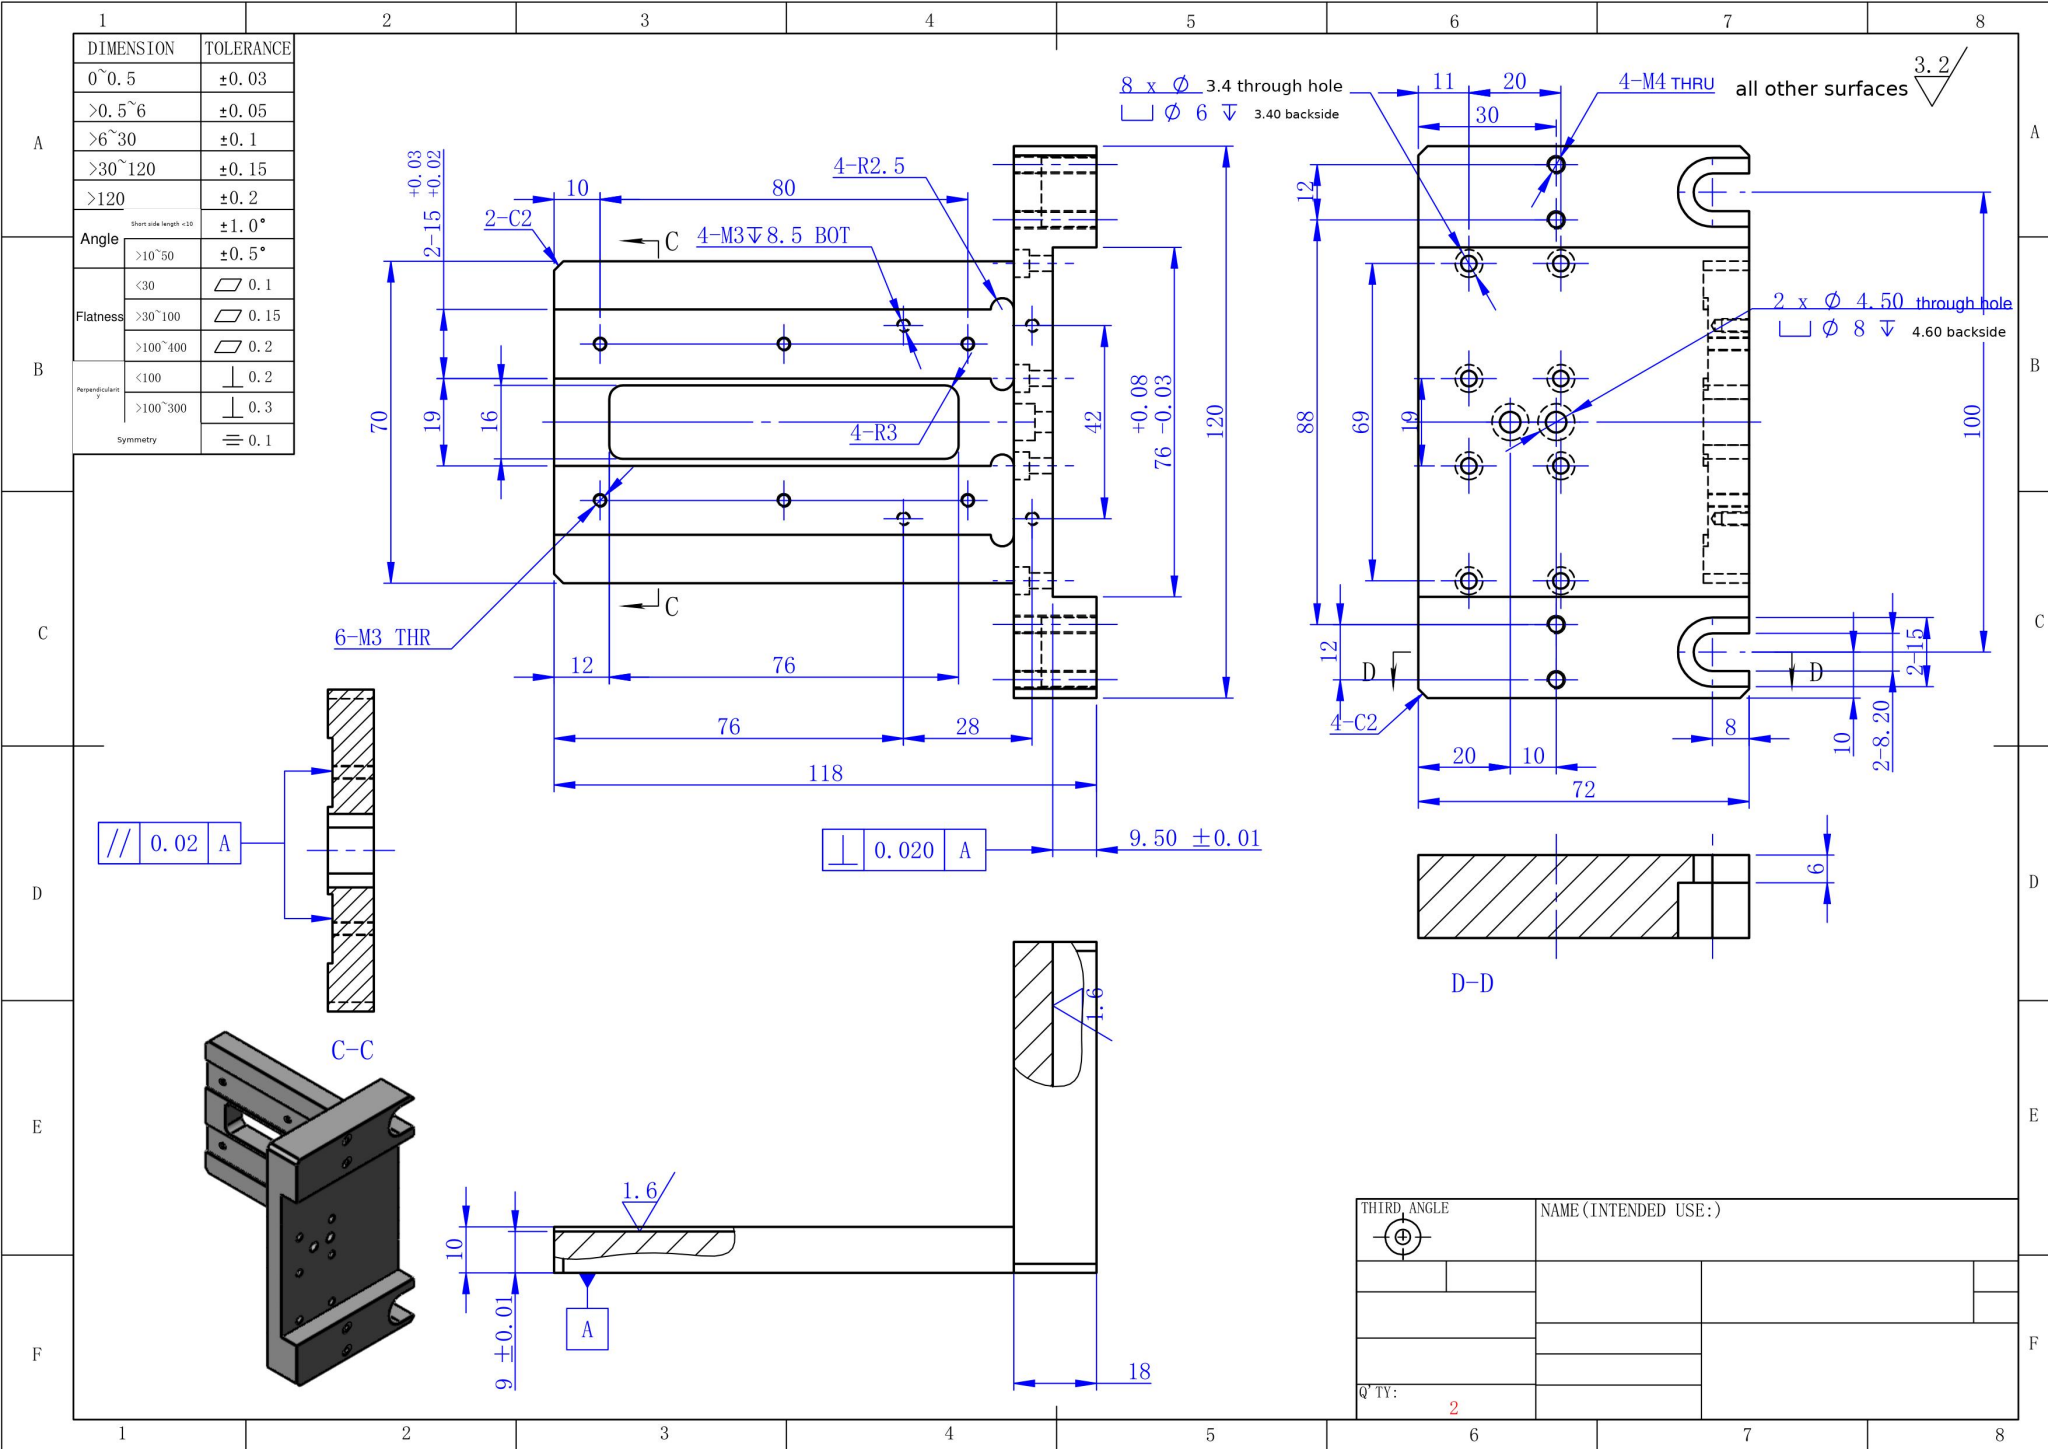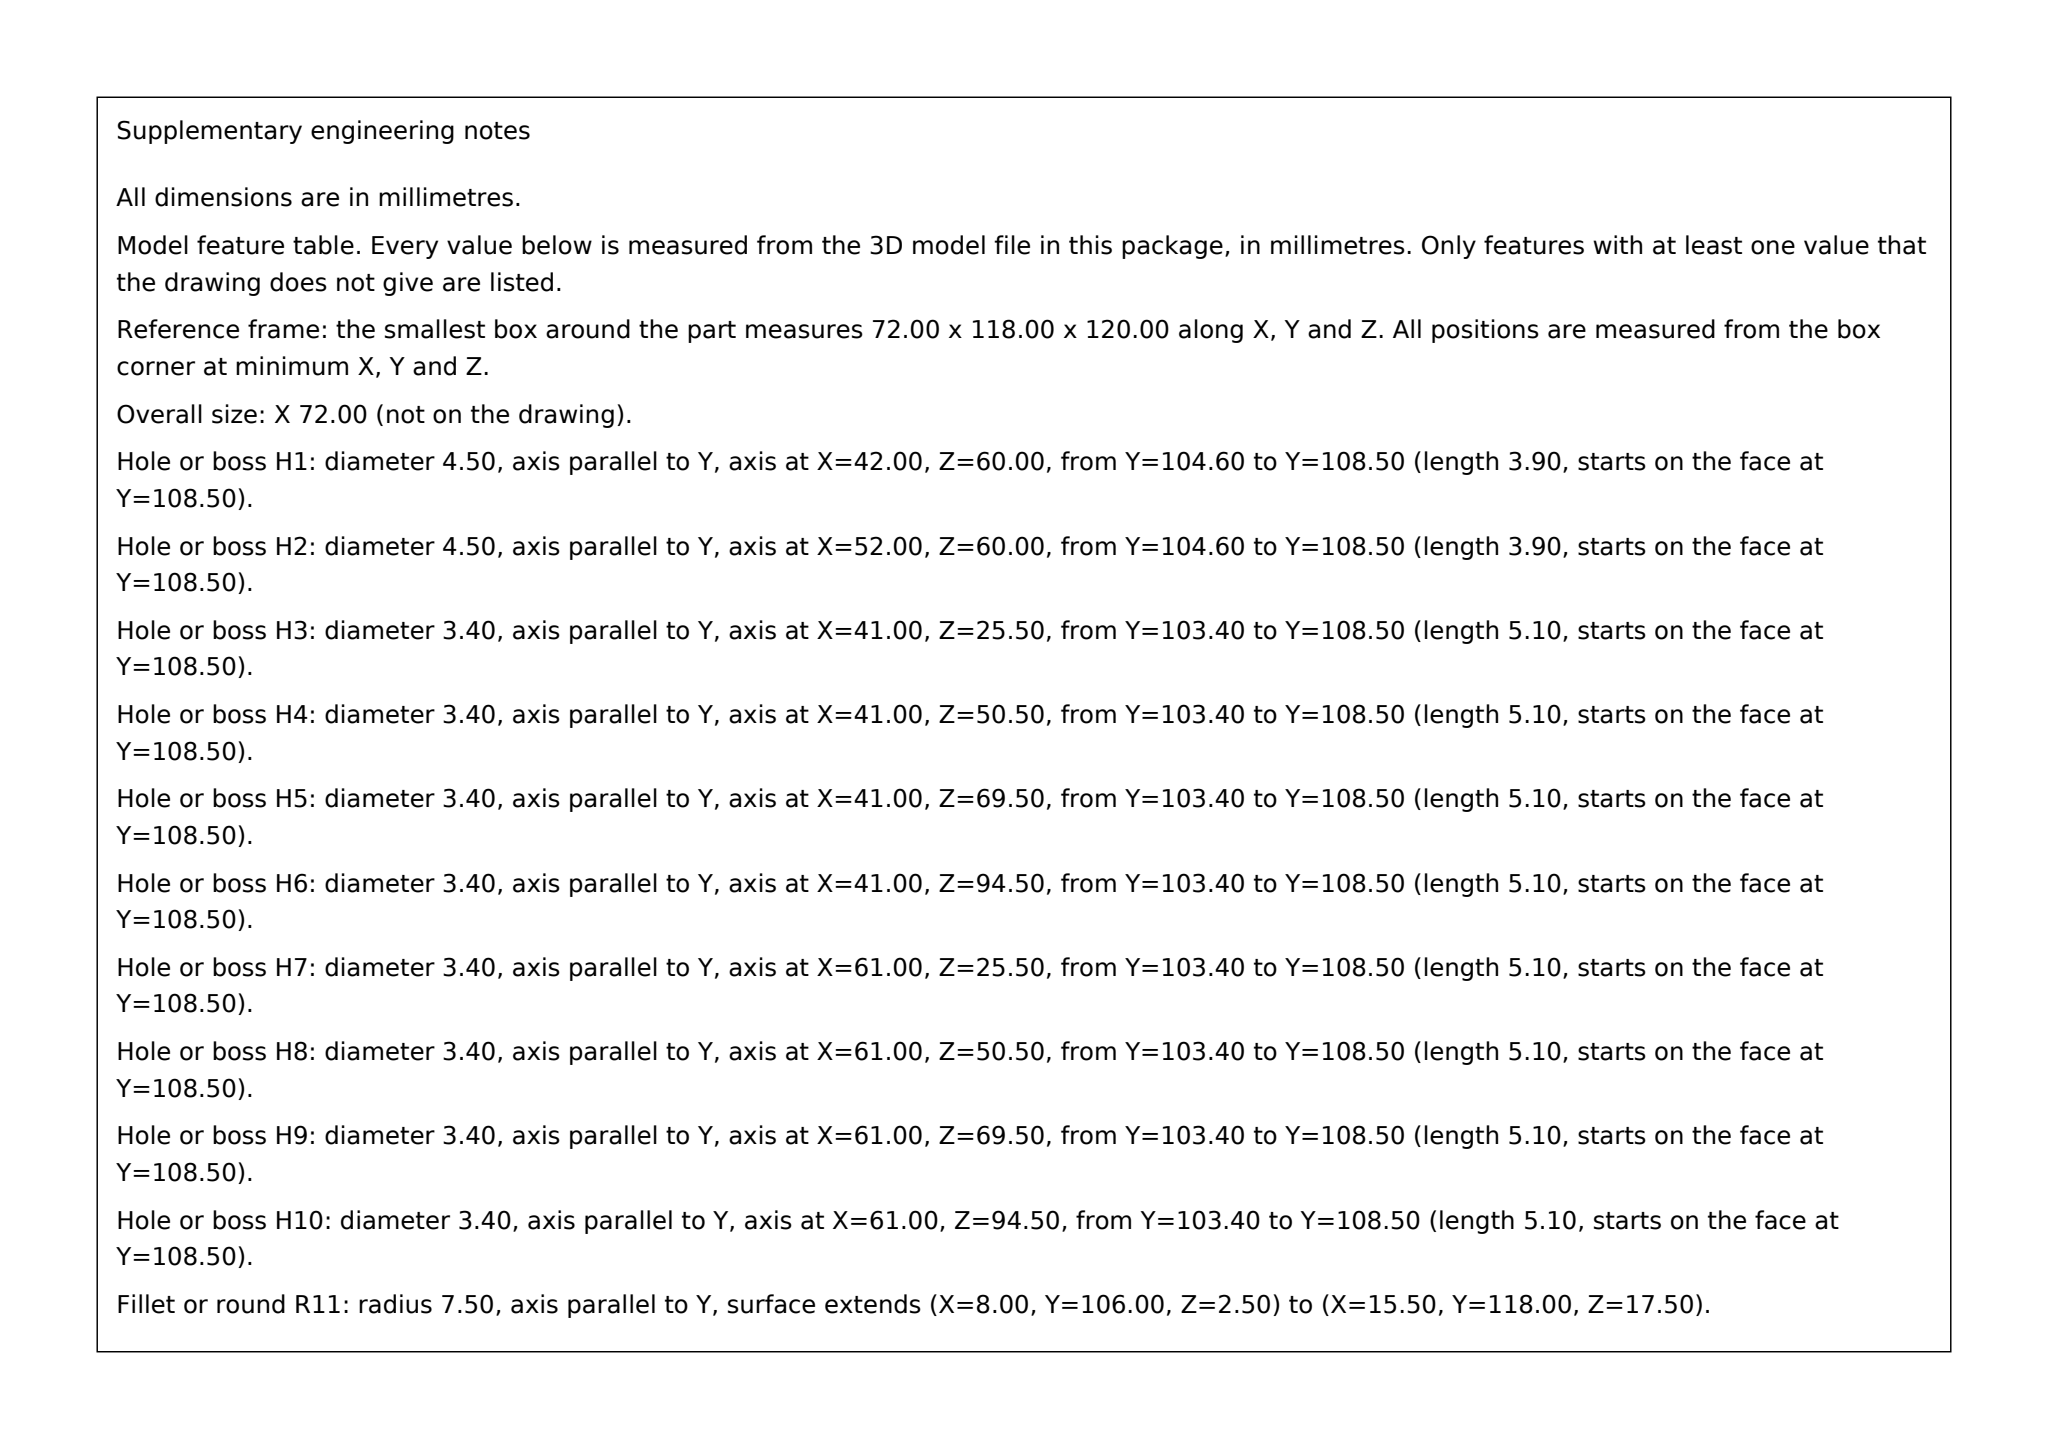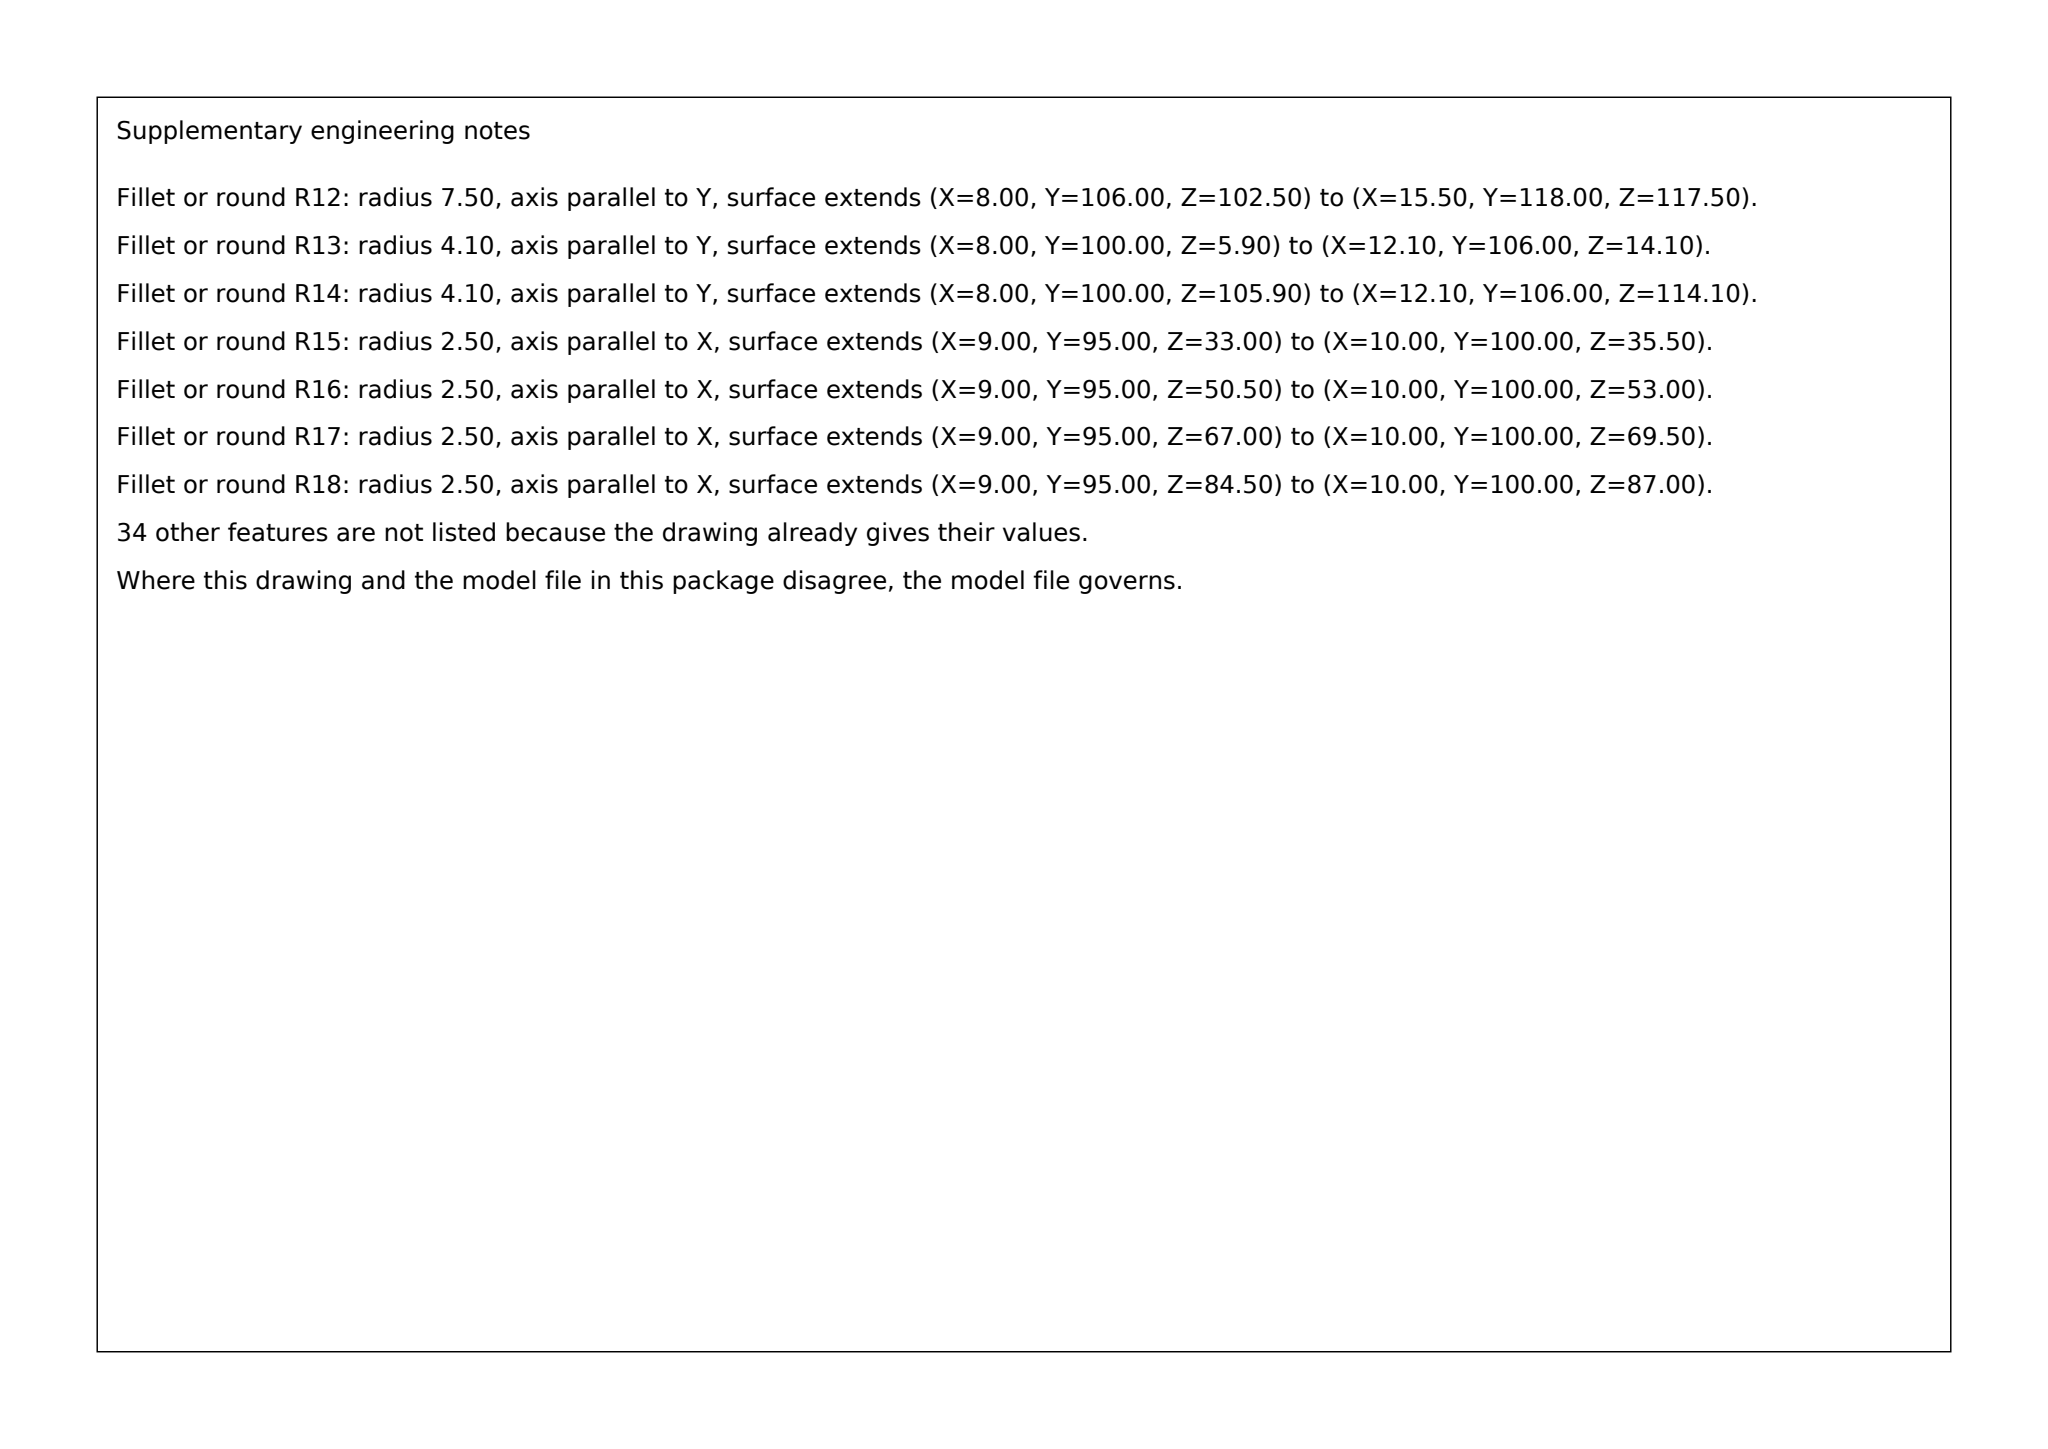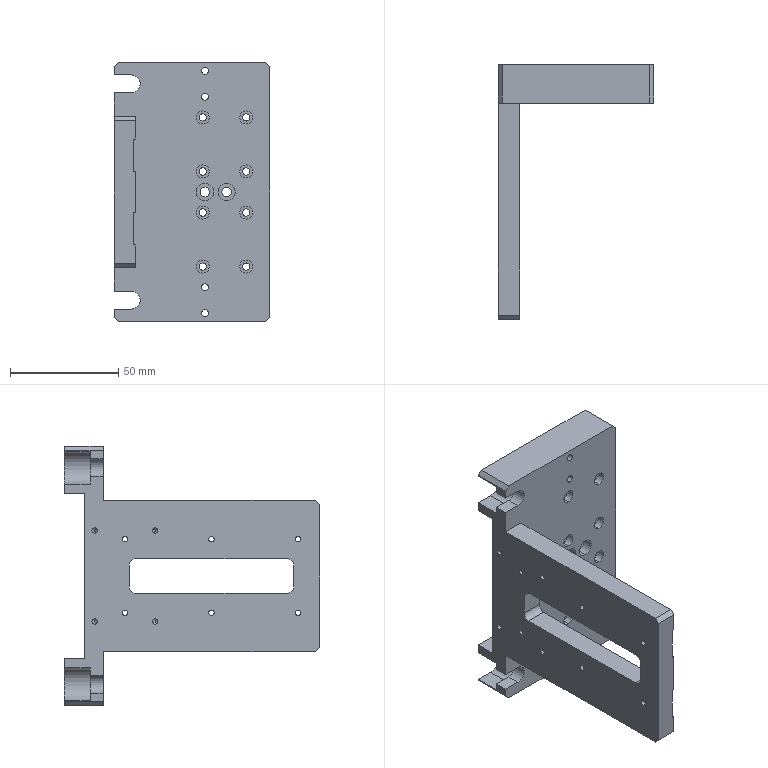Part | SolidWorks | mm | 1 solid | 142 faces | box 72 x 118 x 120 mm | volume 149366 mm3 | cylinder 80 | plane 54 | cone 8 | commonest cylinder face diameters 6 x20 2.5 x20 3.4 x16 3.3 x8 8 x4 4.5 x4 5 x4 8.2 x2
build123d program:
from build123d import *

# Parameters (mm, degrees)
BOSS_EXTRUDE1_DEPTH                                  = 35
SKETCH2_W                                            = 72
SKETCH2_H                                            = 18
BOSS_EXTRUDE2_DEPTH                                  = 25
SKETCH3_W                                            = 16
SKETCH3_H                                            = 76
CUT_EXTRUDE1_DEPTH                                   = 56
FILLET1_R                                            = 3
SKETCH9_W                                            = 21.47
SKETCH9_H                                            = 15
SKETCH9_W_2                                          = 23.046
CUT_EXTRUDE3_DEPTH                                   = 100
SKETCH10_R                                           = 2.5
CUT_EXTRUDE4_DEPTH                                   = 1
M3_TAPPED_HOLE1_D                                    = 2.5
M3_TAPPED_HOLE2_D                                    = 2.5
M3_TAPPED_HOLE2_DEPTH                                = 7.5
M3_TAPPED_HOLE2_TIP                                  = 0.7511
M4_TAPPED_HOLE2_D                                    = 3.3
HOLE_SIZE_ACCORDING_TO_THE_TYPE_OF_HEXAG_D           = 3.4
HOLE_SIZE_ACCORDING_TO_THE_TYPE_OF_HEXAG_CBORE_D     = 6
HOLE_SIZE_ACCORDING_TO_THE_TYPE_OF_HEXAG_CBORE_DEPTH = 3.4
CUT_EXTRUDE6_REACH                                   = 152.692
CUT_EXTRUDE7_DEPTH                                   = 12
CHAMFER1_SIZE                                        = 2
SKETCH23_W                                           = 76
SKETCH23_H                                           = 13.599
CUT_EXTRUDE9_DEPTH                                   = 151.692
HOLE_SIZE_ACCORDING_TO_THE_TYPE_OF_H_2_D             = 4.5
HOLE_SIZE_ACCORDING_TO_THE_TYPE_OF_H_2_CBORE_D       = 8
HOLE_SIZE_ACCORDING_TO_THE_TYPE_OF_H_2_CBORE_DEPTH   = 4.6


with BuildPart() as part:
    # Sketch1 → Boss-Extrude1 (new, symmetric)
    with BuildSketch(Plane.XY):
        Polygon((0, 0), (0, 110), (72, 110), (72, 100), (10, 100), (10, 0), align=None)
    extrude(amount=BOSS_EXTRUDE1_DEPTH, both=True)

    # Sketch2 → Boss-Extrude2 (add)
    with BuildSketch(Plane(origin=(0, 0, -35), x_dir=(-1, 0, 0), z_dir=(0, 0, -1))):
        with Locations((-36, 109)):
            Rectangle(SKETCH2_W, SKETCH2_H)
    boss_extrude2 = extrude(amount=BOSS_EXTRUDE2_DEPTH)

    # Sketch3 → Cut-Extrude1 (cut)
    with BuildSketch(Plane.ZY):
        with Locations((0, 50)):
            Rectangle(SKETCH3_W, SKETCH3_H)
    extrude(amount=-CUT_EXTRUDE1_DEPTH, mode=Mode.SUBTRACT)

    # Fillet1
    fillet1_edges = [part.edges().sort_by_distance(p)[0] for p in [
        (5, 88, 8),
        (5, 12, 8),
        (5, 12, -8),
        (5, 88, -8),
    ]]
    fillet(fillet1_edges, radius=FILLET1_R)

    # Sketch9 → Cut-Extrude3 (cut)
    with BuildSketch(Plane.XZ):
        with Locations((19.735, 17)):
            Rectangle(SKETCH9_W, SKETCH9_H)
        with Locations((20.523, -17)):
            Rectangle(SKETCH9_W_2, SKETCH9_H)
    extrude(amount=-CUT_EXTRUDE3_DEPTH, mode=Mode.SUBTRACT)

    # Sketch10 → Cut-Extrude4 (cut)
    with BuildSketch(Plane(origin=(10, 0, 0), x_dir=(0, 0, -1), z_dir=(1, 0, 0))):
        with Locations((-24.5, 97.5)):
            Circle(SKETCH10_R)
        with Locations((-9.5, 97.5)):
            Circle(SKETCH10_R)
        with Locations((9.5, 97.5)):
            Circle(SKETCH10_R)
        with Locations((24.5, 97.5)):
            Circle(SKETCH10_R)
    extrude(amount=-CUT_EXTRUDE4_DEPTH, mode=Mode.SUBTRACT)

    # M3 Tapped Hole1 (through all)
    with Locations(Plane(origin=(9, 0, 0), x_dir=(0, 0, -1), z_dir=(1, 0, 0))):
        with Locations((-17, 90), (17, 90), (17, 50), (-17, 50), (-17, 10), (17, 10)):
            Hole(M3_TAPPED_HOLE1_D / 2)

    # M3 Tapped Hole2
    with Locations(Plane.ZY):
        with Locations((21, 104), (21, 76), (-21, 104), (-21, 76)):
            Hole(M3_TAPPED_HOLE2_D / 2, depth=M3_TAPPED_HOLE2_DEPTH)
            with Locations((0, 0, -(M3_TAPPED_HOLE2_DEPTH + M3_TAPPED_HOLE2_TIP / 2))):  # 118° drill point
                Cone(0, M3_TAPPED_HOLE2_D / 2, M3_TAPPED_HOLE2_TIP, mode=Mode.SUBTRACT)

    # M4 Tapped Hole2 (through all)
    with Locations(Plane(origin=(6.733, 118, -4.955), x_dir=(1, 0, 0), z_dir=(0, 1, 0))):
        with Locations((35.267, 51.045), (35.267, 39.045)):
            m4_tapped_hole2 = Hole(M4_TAPPED_HOLE2_D / 2)

    # Mirror1: Boss-Extrude2, M4 Tapped Hole2 across plane
    add(boss_extrude2.mirror(Plane.XY))
    add(m4_tapped_hole2.mirror(Plane.XY), mode=Mode.SUBTRACT)

    # Hole Size according to the type of hexag (through all)
    with Locations(Plane(origin=(0, 100, 0), x_dir=(-1, 0, 0), z_dir=(0, -1, 0))):
        with Locations((-41, 34.5), (-61, 34.5), (-41, 9.5), (-61, 9.5), (-41, -9.5), (-41, -34.5), (-61, -34.5), (-61, -9.5)):
            CounterBoreHole(HOLE_SIZE_ACCORDING_TO_THE_TYPE_OF_HEXAG_D / 2, HOLE_SIZE_ACCORDING_TO_THE_TYPE_OF_HEXAG_CBORE_D / 2, HOLE_SIZE_ACCORDING_TO_THE_TYPE_OF_HEXAG_CBORE_DEPTH)

    # Sketch20 → Cut-Extrude6 (cut, up to next)
    with BuildSketch(Plane(origin=(0, 118, 0), x_dir=(1, 0, 0), z_dir=(0, 1, 0)), mode=Mode.PRIVATE) as cut_extrude6_sk1:
        with BuildLine():
            Line((8, 45.9), (0, 45.9))
            ThreePointArc((0, 45.9), (-4.1, 50), (0, 54.1))
            Line((0, 54.1), (8, 54.1))
            ThreePointArc((8, 54.1), (12.1, 50), (8, 45.9))
        make_face()
    cut_extrude6_tool1 = extrude(cut_extrude6_sk1.sketch, amount=-CUT_EXTRUDE6_REACH, mode=Mode.PRIVATE) & part.part
    cut_extrude6 = cut_extrude6_tool1.solids().sort_by_distance((4, 118, -50))[0]
    add(cut_extrude6, mode=Mode.SUBTRACT)

    # Sketch21 → Cut-Extrude7 (cut)
    with BuildSketch(Plane(origin=(0, 118, 0), x_dir=(1, 0, 0), z_dir=(0, 1, 0))):
        with BuildLine():
            Line((8, 42.5), (0, 42.5))
            ThreePointArc((0, 42.5), (-7.5, 50), (0, 57.5))
            Line((0, 57.5), (8, 57.5))
            ThreePointArc((8, 57.5), (15.5, 50), (8, 42.5))
        make_face()
    cut_extrude7 = extrude(amount=-CUT_EXTRUDE7_DEPTH, mode=Mode.SUBTRACT)

    # Chamfer1
    chamfer1_edges = [part.edges().sort_by_distance(p)[0] for p in [
        (72, 109, -60),
        (72, 109, 60),
        (0, 109, 60),
        (0, 109, -60),
        (5, 0, 35),
        (5, 0, -35),
    ]]
    chamfer(chamfer1_edges, length=CHAMFER1_SIZE)

    # Sketch23 → Cut-Extrude9 (cut, through all)
    with BuildSketch(Plane.ZY):
        with Locations((0, 115.299)):
            Rectangle(SKETCH23_W, SKETCH23_H)
    extrude(amount=-CUT_EXTRUDE9_DEPTH, mode=Mode.SUBTRACT)

    # Hole Size according to the type of h 2 (through all)
    with Locations(Plane(origin=(0, 100, 0), x_dir=(-1, 0, 0), z_dir=(0, -1, 0))):
        with Locations((-52, 0), (-42, 0)):
            CounterBoreHole(HOLE_SIZE_ACCORDING_TO_THE_TYPE_OF_H_2_D / 2, HOLE_SIZE_ACCORDING_TO_THE_TYPE_OF_H_2_CBORE_D / 2, HOLE_SIZE_ACCORDING_TO_THE_TYPE_OF_H_2_CBORE_DEPTH)

    # Mirror2: Cut-Extrude6, Cut-Extrude7 across plane
    add(cut_extrude6.mirror(Plane.XY), mode=Mode.SUBTRACT)
    add(cut_extrude7.mirror(Plane.XY), mode=Mode.SUBTRACT)


solid = part.part